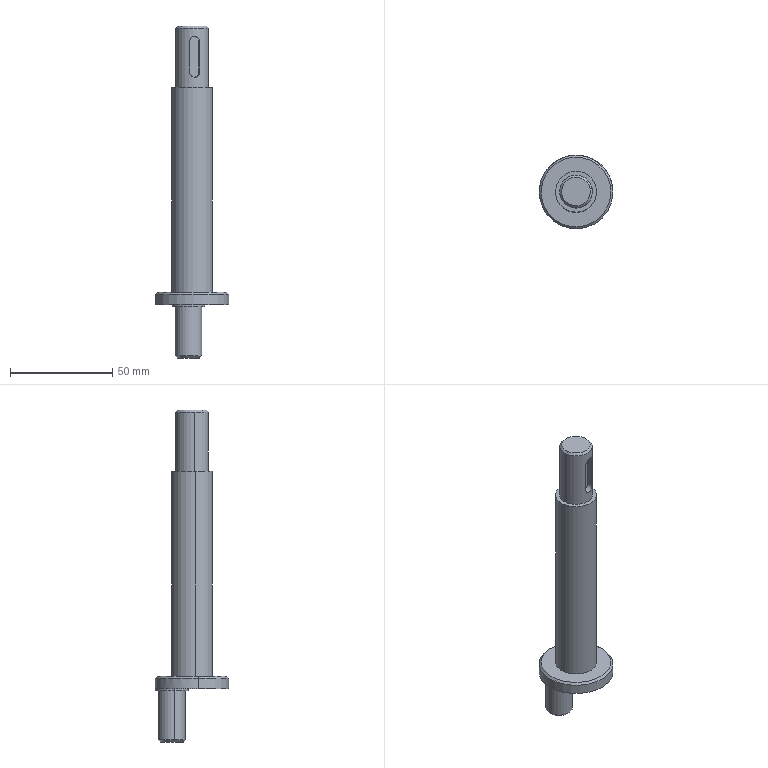Component | SolidWorks | Part5Crankshaft-1 | 1 solid | 27 faces | box 36 x 36 x 162 mm | volume 46703 mm3 | cylinder 12 | plane 9 | cone 6 | commonest cylinder face diameters 16 x4 13 x2 20 x2 36 x2 5 x2
build123d program:
from build123d import *

# Parameters (mm, degrees)
SKETCH1_W           = 30
SKETCH1_H           = 8
SKETCH2_R           = 8
BOSS_EXTRUDE1_DEPTH = 1
SKETCH3_R           = 6.5
BOSS_EXTRUDE2_DEPTH = 25
CHAMFER1_SIZE       = 1
CHAMFER2_SIZE       = 1
CHAMFER3_SIZE       = 1
CUT_EXTRUDE1_DEPTH  = 3


with BuildPart() as part:
    # Sketch1 → Revolve1 (revolve)
    with BuildSketch(Plane.XY, mode=Mode.PRIVATE) as revolve1_sk:
        with Locations((-66, 4)):
            Rectangle(SKETCH1_W, SKETCH1_H)
        Polygon((-51, 8), (-51, 0), (49, 0), (49, 10), (-51, 10), align=None)
        Polygon((49, 10), (49, 0), (55, 0), (55, 18), (49, 18), align=None)
    revolve(revolve1_sk.sketch.rotate(Axis((-81, 0, 0), (1, 0, 0)), 90), axis=Axis((-81, 0, 0), (1, 0, 0)))

    # Sketch2 → Boss-Extrude1 (add)
    with BuildSketch(Plane(origin=(55, 0, 0), x_dir=(0, 0, -1), z_dir=(1, 0, 0))):
        with Locations(Location((0, -10, 0), (0, 0, 270))):
            Circle(SKETCH2_R)
    extrude(amount=BOSS_EXTRUDE1_DEPTH)

    # Sketch3 → Boss-Extrude2 (add)
    with BuildSketch(Plane(origin=(56, 0, 0), x_dir=(0, 0, -1), z_dir=(1, 0, 0))):
        with Locations((0, -10)):
            Circle(SKETCH3_R)
    extrude(amount=BOSS_EXTRUDE2_DEPTH)

    # Chamfer1
    chamfer1_edges = [part.edges().sort_by_distance(p)[0] for p in [
        (81, -10, 6.5),
    ]]
    chamfer(chamfer1_edges, length=CHAMFER1_SIZE)

    # Chamfer2
    chamfer2_edges = [part.edges().sort_by_distance(p)[0] for p in [
        (49, 0, -18),
    ]]
    chamfer(chamfer2_edges, length=CHAMFER2_SIZE)

    # Chamfer3
    chamfer3_edges = [part.edges().sort_by_distance(p)[0] for p in [
        (-81, 0, -8),
    ]]
    chamfer(chamfer3_edges, length=CHAMFER3_SIZE)

    # Sketch6 → Cut-Extrude1 (cut)
    with BuildSketch(Plane(origin=(0, 8, 0), x_dir=(1, 0, 0), z_dir=(0, 1, 0))):
        with BuildLine():
            Line((-73.5, 2.5), (-58.5, 2.5))
            ThreePointArc((-58.5, 2.5), (-56, 0), (-58.5, -2.5))
            Line((-58.5, -2.5), (-73.5, -2.5))
            ThreePointArc((-73.5, -2.5), (-76, 0), (-73.5, 2.5))
        make_face()
    extrude(amount=-CUT_EXTRUDE1_DEPTH, mode=Mode.SUBTRACT)


solid = part.part

# Placed as in the assembly
solid = solid.moved(Location((-80.719, -28.485, 199), (90, -79.746, -90)))
STEP:
#1=COLOUR_RGB('',0.7922,0.8196,0.9333);
#2=FILL_AREA_STYLE_COLOUR('',#1);
#3=FILL_AREA_STYLE('',(#2));
#4=SURFACE_STYLE_FILL_AREA(#3);
#5=SURFACE_SIDE_STYLE('',(#4));
#6=SURFACE_STYLE_USAGE(.BOTH.,#5);
#7=PRESENTATION_STYLE_ASSIGNMENT((#6));
#8=CARTESIAN_POINT('',(-3.449,-1.171,11.024));
#9=VERTEX_POINT('',#8);
#10=CARTESIAN_POINT('',(-2.907,-1.072,11.024));
#11=VERTEX_POINT('',#10);
#12=CARTESIAN_POINT('',(-3.178,-1.121,11.024));
#13=DIRECTION('',(0.,0.,1.));
#14=DIRECTION('',(-0.984,-0.178,0.));
#15=AXIS2_PLACEMENT_3D('',#12,#13,#14);
#16=CIRCLE('',#15,0.2756);
#17=EDGE_CURVE('',#9,#11,#16,.T.);
#18=ORIENTED_EDGE('',*,*,#17,.F.);
#19=CARTESIAN_POINT('',(-3.488,-1.178,10.984));
#20=VERTEX_POINT('',#19);
#21=CARTESIAN_POINT('',(-3.449,-1.171,11.024));
#22=DIRECTION('',(-0.6958,-0.1259,-0.7071));
#23=VECTOR('',#22,39.37);
#24=LINE('',#21,#23);
#25=EDGE_CURVE('',#9,#20,#24,.T.);
#26=ORIENTED_EDGE('',*,*,#25,.T.);
#27=CARTESIAN_POINT('',(-2.868,-1.065,10.984));
#28=VERTEX_POINT('',#27);
#29=CARTESIAN_POINT('',(-3.178,-1.121,10.984));
#30=DIRECTION('',(-0.,-0.,-1.));
#31=DIRECTION('',(-0.984,-0.178,0.));
#32=AXIS2_PLACEMENT_3D('',#29,#30,#31);
#33=CIRCLE('',#32,0.315);
#34=EDGE_CURVE('',#28,#20,#33,.T.);
#35=ORIENTED_EDGE('',*,*,#34,.F.);
#36=CARTESIAN_POINT('',(-2.907,-1.072,11.024));
#37=DIRECTION('',(0.6958,0.1259,-0.7071));
#38=VECTOR('',#37,39.37);
#39=LINE('',#36,#38);
#40=EDGE_CURVE('',#11,#28,#39,.T.);
#41=ORIENTED_EDGE('',*,*,#40,.F.);
#42=EDGE_LOOP('',(#18,#26,#35,#41));
#43=FACE_OUTER_BOUND('',#42,.T.);
#44=CARTESIAN_POINT('',(-3.178,-1.121,11.024));
#45=DIRECTION('',(-0.,-0.,-1.));
#46=DIRECTION('',(0.984,0.178,0.));
#47=AXIS2_PLACEMENT_3D('',#44,#45,#46);
#48=CONICAL_SURFACE('',#47,0.2756,0.7854);
#49=ADVANCED_FACE('',(#43),#48,.T.);
#50=CARTESIAN_POINT('',(-3.837,-1.241,5.906));
#51=VERTEX_POINT('',#50);
#52=CARTESIAN_POINT('',(-2.519,-1.002,5.906));
#53=VERTEX_POINT('',#52);
#54=CARTESIAN_POINT('',(-3.178,-1.121,5.906));
#55=DIRECTION('',(0.,0.,1.));
#56=DIRECTION('',(0.984,0.178,0.));
#57=AXIS2_PLACEMENT_3D('',#54,#55,#56);
#58=CIRCLE('',#57,0.6693);
#59=EDGE_CURVE('',#51,#53,#58,.T.);
#60=ORIENTED_EDGE('',*,*,#59,.F.);
#61=CARTESIAN_POINT('',(-3.875,-1.248,5.866));
#62=VERTEX_POINT('',#61);
#63=CARTESIAN_POINT('',(-3.837,-1.241,5.906));
#64=DIRECTION('',(-0.6958,-0.1259,-0.7071));
#65=VECTOR('',#64,39.37);
#66=LINE('',#63,#65);
#67=EDGE_CURVE('',#51,#62,#66,.T.);
#68=ORIENTED_EDGE('',*,*,#67,.T.);
#69=CARTESIAN_POINT('',(-2.481,-0.9953,5.866));
#70=VERTEX_POINT('',#69);
#71=CARTESIAN_POINT('',(-3.178,-1.121,5.866));
#72=DIRECTION('',(-0.,-0.,-1.));
#73=DIRECTION('',(0.984,0.178,0.));
#74=AXIS2_PLACEMENT_3D('',#71,#72,#73);
#75=CIRCLE('',#74,0.7087);
#76=EDGE_CURVE('',#70,#62,#75,.T.);
#77=ORIENTED_EDGE('',*,*,#76,.F.);
#78=CARTESIAN_POINT('',(-2.519,-1.002,5.906));
#79=DIRECTION('',(0.6958,0.1259,-0.7071));
#80=VECTOR('',#79,39.37);
#81=LINE('',#78,#80);
#82=EDGE_CURVE('',#53,#70,#81,.T.);
#83=ORIENTED_EDGE('',*,*,#82,.F.);
#84=EDGE_LOOP('',(#60,#68,#77,#83));
#85=FACE_OUTER_BOUND('',#84,.T.);
#86=CARTESIAN_POINT('',(-3.178,-1.121,5.906));
#87=DIRECTION('',(-0.,-0.,-1.));
#88=DIRECTION('',(0.984,0.178,0.));
#89=AXIS2_PLACEMENT_3D('',#86,#87,#88);
#90=CONICAL_SURFACE('',#89,0.6693,0.7854);
#91=ADVANCED_FACE('',(#85),#90,.T.);
#92=CARTESIAN_POINT('',(-3.035,-0.6955,4.646));
#93=VERTEX_POINT('',#92);
#94=CARTESIAN_POINT('',(-3.461,-0.7726,4.646));
#95=VERTEX_POINT('',#94);
#96=CARTESIAN_POINT('',(-3.248,-0.7341,4.646));
#97=DIRECTION('',(-0.,-0.,-1.));
#98=DIRECTION('',(0.984,0.178,0.));
#99=AXIS2_PLACEMENT_3D('',#96,#97,#98);
#100=CIRCLE('',#99,0.2165);
#101=EDGE_CURVE('',#93,#95,#100,.T.);
#102=ORIENTED_EDGE('',*,*,#101,.F.);
#103=CARTESIAN_POINT('',(-2.996,-0.6885,4.685));
#104=VERTEX_POINT('',#103);
#105=CARTESIAN_POINT('',(-3.035,-0.6955,4.646));
#106=DIRECTION('',(0.6958,0.1259,0.7071));
#107=VECTOR('',#106,39.37);
#108=LINE('',#105,#107);
#109=EDGE_CURVE('',#93,#104,#108,.T.);
#110=ORIENTED_EDGE('',*,*,#109,.T.);
#111=CARTESIAN_POINT('',(-3.5,-0.7796,4.685));
#112=VERTEX_POINT('',#111);
#113=CARTESIAN_POINT('',(-3.248,-0.7341,4.685));
#114=DIRECTION('',(0.,0.,1.));
#115=DIRECTION('',(0.984,0.178,0.));
#116=AXIS2_PLACEMENT_3D('',#113,#114,#115);
#117=CIRCLE('',#116,0.2559);
#118=EDGE_CURVE('',#112,#104,#117,.T.);
#119=ORIENTED_EDGE('',*,*,#118,.F.);
#120=CARTESIAN_POINT('',(-3.461,-0.7726,4.646));
#121=DIRECTION('',(-0.6958,-0.1259,0.7071));
#122=VECTOR('',#121,39.37);
#123=LINE('',#120,#122);
#124=EDGE_CURVE('',#95,#112,#123,.T.);
#125=ORIENTED_EDGE('',*,*,#124,.F.);
#126=EDGE_LOOP('',(#102,#110,#119,#125));
#127=FACE_OUTER_BOUND('',#126,.T.);
#128=CARTESIAN_POINT('',(-3.248,-0.7341,4.646));
#129=DIRECTION('',(0.,0.,1.));
#130=DIRECTION('',(-0.984,-0.178,0.));
#131=AXIS2_PLACEMENT_3D('',#128,#129,#130);
#132=CONICAL_SURFACE('',#131,0.2165,0.7854);
#133=ADVANCED_FACE('',(#127),#132,.T.);
#134=ORIENTED_EDGE('',*,*,#118,.T.);
#135=CARTESIAN_POINT('',(-2.996,-0.6885,5.63));
#136=VERTEX_POINT('',#135);
#137=CARTESIAN_POINT('',(-2.996,-0.6885,4.646));
#138=DIRECTION('',(0.,0.,1.));
#139=VECTOR('',#138,39.37);
#140=LINE('',#137,#139);
#141=EDGE_CURVE('',#104,#136,#140,.T.);
#142=ORIENTED_EDGE('',*,*,#141,.T.);
#143=CARTESIAN_POINT('',(-3.5,-0.7796,5.63));
#144=VERTEX_POINT('',#143);
#145=CARTESIAN_POINT('',(-3.248,-0.7341,5.63));
#146=DIRECTION('',(-0.,-0.,-1.));
#147=DIRECTION('',(0.984,0.178,0.));
#148=AXIS2_PLACEMENT_3D('',#145,#146,#147);
#149=CIRCLE('',#148,0.2559);
#150=EDGE_CURVE('',#136,#144,#149,.T.);
#151=ORIENTED_EDGE('',*,*,#150,.T.);
#152=CARTESIAN_POINT('',(-3.5,-0.7796,4.646));
#153=DIRECTION('',(0.,0.,1.));
#154=VECTOR('',#153,39.37);
#155=LINE('',#152,#154);
#156=EDGE_CURVE('',#112,#144,#155,.T.);
#157=ORIENTED_EDGE('',*,*,#156,.F.);
#158=EDGE_LOOP('',(#134,#142,#151,#157));
#159=FACE_OUTER_BOUND('',#158,.T.);
#160=CARTESIAN_POINT('',(-3.248,-0.7341,4.646));
#161=DIRECTION('',(0.,0.,1.));
#162=DIRECTION('',(-0.984,-0.178,0.));
#163=AXIS2_PLACEMENT_3D('',#160,#161,#162);
#164=CYLINDRICAL_SURFACE('',#163,0.2559);
#165=ADVANCED_FACE('',(#159),#164,.T.);
#166=CARTESIAN_POINT('',(-2.938,-0.678,5.63));
#167=VERTEX_POINT('',#166);
#168=CARTESIAN_POINT('',(-3.558,-0.7901,5.63));
#169=VERTEX_POINT('',#168);
#170=CARTESIAN_POINT('',(-3.248,-0.7341,5.63));
#171=DIRECTION('',(-0.,-0.,-1.));
#172=DIRECTION('',(0.984,0.178,0.));
#173=AXIS2_PLACEMENT_3D('',#170,#171,#172);
#174=CIRCLE('',#173,0.315);
#175=EDGE_CURVE('',#167,#169,#174,.T.);
#176=ORIENTED_EDGE('',*,*,#175,.F.);
#177=CARTESIAN_POINT('',(-2.938,-0.678,5.669));
#178=VERTEX_POINT('',#177);
#179=CARTESIAN_POINT('',(-2.938,-0.678,5.63));
#180=DIRECTION('',(0.,0.,1.));
#181=VECTOR('',#180,39.37);
#182=LINE('',#179,#181);
#183=EDGE_CURVE('',#167,#178,#182,.T.);
#184=ORIENTED_EDGE('',*,*,#183,.T.);
#185=CARTESIAN_POINT('',(-3.558,-0.7901,5.669));
#186=VERTEX_POINT('',#185);
#187=CARTESIAN_POINT('',(-3.248,-0.7341,5.669));
#188=DIRECTION('',(-0.,-0.,-1.));
#189=DIRECTION('',(0.984,0.178,0.));
#190=AXIS2_PLACEMENT_3D('',#187,#188,#189);
#191=CIRCLE('',#190,0.315);
#192=EDGE_CURVE('',#178,#186,#191,.T.);
#193=ORIENTED_EDGE('',*,*,#192,.T.);
#194=CARTESIAN_POINT('',(-3.558,-0.7901,5.63));
#195=DIRECTION('',(0.,0.,1.));
#196=VECTOR('',#195,39.37);
#197=LINE('',#194,#196);
#198=EDGE_CURVE('',#169,#186,#197,.T.);
#199=ORIENTED_EDGE('',*,*,#198,.F.);
#200=EDGE_LOOP('',(#176,#184,#193,#199));
#201=FACE_OUTER_BOUND('',#200,.T.);
#202=CARTESIAN_POINT('',(-3.248,-0.7341,5.63));
#203=DIRECTION('',(0.,0.,1.));
#204=DIRECTION('',(-0.984,-0.178,0.));
#205=AXIS2_PLACEMENT_3D('',#202,#203,#204);
#206=CYLINDRICAL_SURFACE('',#205,0.315);
#207=ADVANCED_FACE('',(#201),#206,.T.);
#208=CARTESIAN_POINT('',(-3.222,-1.433,10.138));
#209=VERTEX_POINT('',#208);
#210=CARTESIAN_POINT('',(-3.028,-1.398,10.138));
#211=VERTEX_POINT('',#210);
#212=CARTESIAN_POINT('',(-3.222,-1.433,10.138));
#213=CARTESIAN_POINT('',(-3.222,-1.433,10.131));
#214=CARTESIAN_POINT('',(-3.221,-1.433,10.125));
#215=CARTESIAN_POINT('',(-3.218,-1.434,10.112));
#216=CARTESIAN_POINT('',(-3.216,-1.434,10.106));
#217=CARTESIAN_POINT('',(-3.211,-1.435,10.094));
#218=CARTESIAN_POINT('',(-3.208,-1.435,10.088));
#219=CARTESIAN_POINT('',(-3.201,-1.436,10.078));
#220=CARTESIAN_POINT('',(-3.196,-1.436,10.073));
#221=CARTESIAN_POINT('',(-3.182,-1.437,10.059));
#222=CARTESIAN_POINT('',(-3.171,-1.437,10.052));
#223=CARTESIAN_POINT('',(-3.154,-1.436,10.044));
#224=CARTESIAN_POINT('',(-3.147,-1.435,10.043));
#225=CARTESIAN_POINT('',(-3.135,-1.434,10.04));
#226=CARTESIAN_POINT('',(-3.128,-1.433,10.039));
#227=CARTESIAN_POINT('',(-3.116,-1.43,10.039));
#228=CARTESIAN_POINT('',(-3.109,-1.429,10.04));
#229=CARTESIAN_POINT('',(-3.097,-1.426,10.043));
#230=CARTESIAN_POINT('',(-3.091,-1.424,10.044));
#231=CARTESIAN_POINT('',(-3.079,-1.421,10.049));
#232=CARTESIAN_POINT('',(-3.074,-1.419,10.052));
#233=CARTESIAN_POINT('',(-3.064,-1.415,10.06));
#234=CARTESIAN_POINT('',(-3.059,-1.413,10.064));
#235=CARTESIAN_POINT('',(-3.05,-1.41,10.073));
#236=CARTESIAN_POINT('',(-3.047,-1.408,10.078));
#237=CARTESIAN_POINT('',(-3.04,-1.405,10.088));
#238=CARTESIAN_POINT('',(-3.037,-1.403,10.094));
#239=CARTESIAN_POINT('',(-3.033,-1.401,10.106));
#240=CARTESIAN_POINT('',(-3.031,-1.4,10.112));
#241=CARTESIAN_POINT('',(-3.028,-1.399,10.125));
#242=CARTESIAN_POINT('',(-3.028,-1.398,10.131));
#243=CARTESIAN_POINT('',(-3.028,-1.398,10.138));
#244=B_SPLINE_CURVE_WITH_KNOTS('',3,(#212,#213,#214,#215,#216,#217,#218,#219,#220,#221,#222,#223,#224,#225,#226,#227,#228,#229,#230,#231,#232,#233,#234,#235,#236,#237,#238,#239,#240,#241,#242,#243),.UNSPECIFIED.,.F.,.F.,(4,2,2,2,2,2,2,2,2,2,2,2,2,2,2,4),(0.,0.0004914,0.0009828,0.001474,0.001966,0.002949,0.00344,0.003931,0.004423,0.004914,0.005406,0.005897,0.006388,0.00688,0.007371,0.007863),.UNSPECIFIED.);
#245=EDGE_CURVE('',#209,#211,#244,.T.);
#246=ORIENTED_EDGE('',*,*,#245,.F.);
#247=CARTESIAN_POINT('',(-3.222,-1.433,10.728));
#248=VERTEX_POINT('',#247);
#249=CARTESIAN_POINT('',(-3.222,-1.433,11.024));
#250=DIRECTION('',(-0.,-0.,-1.));
#251=VECTOR('',#250,39.37);
#252=LINE('',#249,#251);
#253=EDGE_CURVE('',#248,#209,#252,.T.);
#254=ORIENTED_EDGE('',*,*,#253,.F.);
#255=CARTESIAN_POINT('',(-3.028,-1.398,10.728));
#256=VERTEX_POINT('',#255);
#257=CARTESIAN_POINT('',(-3.028,-1.398,10.728));
#258=CARTESIAN_POINT('',(-3.028,-1.398,10.735));
#259=CARTESIAN_POINT('',(-3.028,-1.399,10.741));
#260=CARTESIAN_POINT('',(-3.031,-1.4,10.754));
#261=CARTESIAN_POINT('',(-3.033,-1.401,10.76));
#262=CARTESIAN_POINT('',(-3.037,-1.403,10.772));
#263=CARTESIAN_POINT('',(-3.04,-1.405,10.778));
#264=CARTESIAN_POINT('',(-3.047,-1.408,10.788));
#265=CARTESIAN_POINT('',(-3.05,-1.41,10.793));
#266=CARTESIAN_POINT('',(-3.063,-1.415,10.807));
#267=CARTESIAN_POINT('',(-3.074,-1.419,10.814));
#268=CARTESIAN_POINT('',(-3.091,-1.424,10.822));
#269=CARTESIAN_POINT('',(-3.097,-1.426,10.824));
#270=CARTESIAN_POINT('',(-3.109,-1.429,10.826));
#271=CARTESIAN_POINT('',(-3.115,-1.43,10.827));
#272=CARTESIAN_POINT('',(-3.128,-1.433,10.827));
#273=CARTESIAN_POINT('',(-3.135,-1.434,10.826));
#274=CARTESIAN_POINT('',(-3.147,-1.435,10.824));
#275=CARTESIAN_POINT('',(-3.153,-1.436,10.822));
#276=CARTESIAN_POINT('',(-3.165,-1.436,10.817));
#277=CARTESIAN_POINT('',(-3.171,-1.436,10.814));
#278=CARTESIAN_POINT('',(-3.182,-1.436,10.807));
#279=CARTESIAN_POINT('',(-3.187,-1.436,10.802));
#280=CARTESIAN_POINT('',(-3.196,-1.436,10.793));
#281=CARTESIAN_POINT('',(-3.201,-1.436,10.789));
#282=CARTESIAN_POINT('',(-3.208,-1.435,10.778));
#283=CARTESIAN_POINT('',(-3.211,-1.435,10.772));
#284=CARTESIAN_POINT('',(-3.216,-1.434,10.76));
#285=CARTESIAN_POINT('',(-3.218,-1.434,10.754));
#286=CARTESIAN_POINT('',(-3.221,-1.433,10.741));
#287=CARTESIAN_POINT('',(-3.222,-1.433,10.735));
#288=CARTESIAN_POINT('',(-3.222,-1.433,10.728));
#289=B_SPLINE_CURVE_WITH_KNOTS('',3,(#257,#258,#259,#260,#261,#262,#263,#264,#265,#266,#267,#268,#269,#270,#271,#272,#273,#274,#275,#276,#277,#278,#279,#280,#281,#282,#283,#284,#285,#286,#287,#288),.UNSPECIFIED.,.F.,.F.,(4,2,2,2,2,2,2,2,2,2,2,2,2,2,2,4),(0.,0.0004914,0.0009828,0.001474,0.001966,0.002949,0.00344,0.003931,0.004423,0.004914,0.005406,0.005897,0.006388,0.00688,0.007371,0.007863),.UNSPECIFIED.);
#290=EDGE_CURVE('',#256,#248,#289,.T.);
#291=ORIENTED_EDGE('',*,*,#290,.F.);
#292=CARTESIAN_POINT('',(-3.028,-1.398,11.024));
#293=DIRECTION('',(0.,0.,1.));
#294=VECTOR('',#293,39.37);
#295=LINE('',#292,#294);
#296=EDGE_CURVE('',#211,#256,#295,.T.);
#297=ORIENTED_EDGE('',*,*,#296,.F.);
#298=EDGE_LOOP('',(#246,#254,#291,#297));
#299=FACE_BOUND('',#298,.T.);
#300=CARTESIAN_POINT('',(-3.488,-1.178,9.843));
#301=VERTEX_POINT('',#300);
#302=CARTESIAN_POINT('',(-2.868,-1.065,9.843));
#303=VERTEX_POINT('',#302);
#304=CARTESIAN_POINT('',(-3.178,-1.121,9.843));
#305=DIRECTION('',(0.,0.,1.));
#306=DIRECTION('',(-0.984,-0.178,0.));
#307=AXIS2_PLACEMENT_3D('',#304,#305,#306);
#308=CIRCLE('',#307,0.315);
#309=EDGE_CURVE('',#301,#303,#308,.T.);
#310=ORIENTED_EDGE('',*,*,#309,.T.);
#311=CARTESIAN_POINT('',(-2.868,-1.065,11.024));
#312=DIRECTION('',(0.,0.,1.));
#313=VECTOR('',#312,39.37);
#314=LINE('',#311,#313);
#315=EDGE_CURVE('',#303,#28,#314,.T.);
#316=ORIENTED_EDGE('',*,*,#315,.T.);
#317=ORIENTED_EDGE('',*,*,#34,.T.);
#318=CARTESIAN_POINT('',(-3.488,-1.178,11.024));
#319=DIRECTION('',(0.,0.,1.));
#320=VECTOR('',#319,39.37);
#321=LINE('',#318,#320);
#322=EDGE_CURVE('',#301,#20,#321,.T.);
#323=ORIENTED_EDGE('',*,*,#322,.F.);
#324=EDGE_LOOP('',(#310,#316,#317,#323));
#325=FACE_OUTER_BOUND('',#324,.T.);
#326=CARTESIAN_POINT('',(-3.178,-1.121,11.024));
#327=DIRECTION('',(0.,0.,1.));
#328=DIRECTION('',(-0.984,-0.178,0.));
#329=AXIS2_PLACEMENT_3D('',#326,#327,#328);
#330=CYLINDRICAL_SURFACE('',#329,0.315);
#331=ADVANCED_FACE('',(#299,#325),#330,.T.);
#332=CARTESIAN_POINT('',(-3.565,-1.192,5.906));
#333=VERTEX_POINT('',#332);
#334=CARTESIAN_POINT('',(-2.79,-1.051,5.906));
#335=VERTEX_POINT('',#334);
#336=CARTESIAN_POINT('',(-3.178,-1.121,5.906));
#337=DIRECTION('',(0.,0.,1.));
#338=DIRECTION('',(-0.984,-0.178,0.));
#339=AXIS2_PLACEMENT_3D('',#336,#337,#338);
#340=CIRCLE('',#339,0.3937);
#341=EDGE_CURVE('',#333,#335,#340,.T.);
#342=ORIENTED_EDGE('',*,*,#341,.T.);
#343=CARTESIAN_POINT('',(-2.79,-1.051,9.843));
#344=VERTEX_POINT('',#343);
#345=CARTESIAN_POINT('',(-2.79,-1.051,11.024));
#346=DIRECTION('',(0.,0.,1.));
#347=VECTOR('',#346,39.37);
#348=LINE('',#345,#347);
#349=EDGE_CURVE('',#335,#344,#348,.T.);
#350=ORIENTED_EDGE('',*,*,#349,.T.);
#351=CARTESIAN_POINT('',(-3.565,-1.192,9.843));
#352=VERTEX_POINT('',#351);
#353=CARTESIAN_POINT('',(-3.178,-1.121,9.843));
#354=DIRECTION('',(0.,0.,1.));
#355=DIRECTION('',(-0.984,-0.178,0.));
#356=AXIS2_PLACEMENT_3D('',#353,#354,#355);
#357=CIRCLE('',#356,0.3937);
#358=EDGE_CURVE('',#352,#344,#357,.T.);
#359=ORIENTED_EDGE('',*,*,#358,.F.);
#360=CARTESIAN_POINT('',(-3.565,-1.192,11.024));
#361=DIRECTION('',(0.,0.,1.));
#362=VECTOR('',#361,39.37);
#363=LINE('',#360,#362);
#364=EDGE_CURVE('',#333,#352,#363,.T.);
#365=ORIENTED_EDGE('',*,*,#364,.F.);
#366=EDGE_LOOP('',(#342,#350,#359,#365));
#367=FACE_OUTER_BOUND('',#366,.T.);
#368=CARTESIAN_POINT('',(-3.178,-1.121,11.024));
#369=DIRECTION('',(0.,0.,1.));
#370=DIRECTION('',(-0.984,-0.178,0.));
#371=AXIS2_PLACEMENT_3D('',#368,#369,#370);
#372=CYLINDRICAL_SURFACE('',#371,0.3937);
#373=ADVANCED_FACE('',(#367),#372,.T.);
#374=CARTESIAN_POINT('',(-3.875,-1.248,5.669));
#375=VERTEX_POINT('',#374);
#376=CARTESIAN_POINT('',(-2.481,-0.9953,5.669));
#377=VERTEX_POINT('',#376);
#378=CARTESIAN_POINT('',(-3.178,-1.121,5.669));
#379=DIRECTION('',(0.,0.,1.));
#380=DIRECTION('',(-0.984,-0.178,0.));
#381=AXIS2_PLACEMENT_3D('',#378,#379,#380);
#382=CIRCLE('',#381,0.7087);
#383=EDGE_CURVE('',#375,#377,#382,.T.);
#384=ORIENTED_EDGE('',*,*,#383,.T.);
#385=CARTESIAN_POINT('',(-2.481,-0.9953,11.024));
#386=DIRECTION('',(0.,0.,1.));
#387=VECTOR('',#386,39.37);
#388=LINE('',#385,#387);
#389=EDGE_CURVE('',#377,#70,#388,.T.);
#390=ORIENTED_EDGE('',*,*,#389,.T.);
#391=ORIENTED_EDGE('',*,*,#76,.T.);
#392=CARTESIAN_POINT('',(-3.875,-1.248,11.024));
#393=DIRECTION('',(0.,0.,1.));
#394=VECTOR('',#393,39.37);
#395=LINE('',#392,#394);
#396=EDGE_CURVE('',#375,#62,#395,.T.);
#397=ORIENTED_EDGE('',*,*,#396,.F.);
#398=EDGE_LOOP('',(#384,#390,#391,#397));
#399=FACE_OUTER_BOUND('',#398,.T.);
#400=CARTESIAN_POINT('',(-3.178,-1.121,11.024));
#401=DIRECTION('',(0.,0.,1.));
#402=DIRECTION('',(-0.984,-0.178,0.));
#403=AXIS2_PLACEMENT_3D('',#400,#401,#402);
#404=CYLINDRICAL_SURFACE('',#403,0.7087);
#405=ADVANCED_FACE('',(#399),#404,.T.);
#406=CARTESIAN_POINT('',(-3.178,-1.121,11.024));
#407=DIRECTION('',(0.,0.,1.));
#408=DIRECTION('',(-0.984,-0.178,0.));
#409=AXIS2_PLACEMENT_3D('',#406,#407,#408);
#410=CIRCLE('',#409,0.2756);
#411=EDGE_CURVE('',#11,#9,#410,.T.);
#412=ORIENTED_EDGE('',*,*,#411,.T.);
#413=ORIENTED_EDGE('',*,*,#17,.T.);
#414=EDGE_LOOP('',(#412,#413));
#415=FACE_OUTER_BOUND('',#414,.T.);
#416=CARTESIAN_POINT('',(-3.178,-1.121,11.024));
#417=DIRECTION('',(0.,0.,1.));
#418=DIRECTION('',(-0.984,-0.178,0.));
#419=AXIS2_PLACEMENT_3D('',#416,#417,#418);
#420=PLANE('',#419);
#421=ADVANCED_FACE('',(#415),#420,.T.);
#422=CARTESIAN_POINT('',(-3.304,-0.4241,5.669));
#423=VERTEX_POINT('',#422);
#424=CARTESIAN_POINT('',(-3.178,-1.121,5.669));
#425=DIRECTION('',(0.,0.,1.));
#426=DIRECTION('',(-0.984,-0.178,0.));
#427=AXIS2_PLACEMENT_3D('',#424,#425,#426);
#428=CIRCLE('',#427,0.7087);
#429=EDGE_CURVE('',#423,#375,#428,.T.);
#430=ORIENTED_EDGE('',*,*,#429,.F.);
#431=CARTESIAN_POINT('',(-3.248,-0.7341,5.669));
#432=DIRECTION('',(-0.,-0.,-1.));
#433=DIRECTION('',(0.984,0.178,0.));
#434=AXIS2_PLACEMENT_3D('',#431,#432,#433);
#435=CIRCLE('',#434,0.315);
#436=EDGE_CURVE('',#186,#423,#435,.T.);
#437=ORIENTED_EDGE('',*,*,#436,.F.);
#438=ORIENTED_EDGE('',*,*,#192,.F.);
#439=CARTESIAN_POINT('',(-3.248,-0.7341,5.669));
#440=DIRECTION('',(-0.,-0.,-1.));
#441=DIRECTION('',(0.984,0.178,0.));
#442=AXIS2_PLACEMENT_3D('',#439,#440,#441);
#443=CIRCLE('',#442,0.315);
#444=EDGE_CURVE('',#423,#178,#443,.T.);
#445=ORIENTED_EDGE('',*,*,#444,.F.);
#446=CARTESIAN_POINT('',(-3.178,-1.121,5.669));
#447=DIRECTION('',(0.,0.,1.));
#448=DIRECTION('',(-0.984,-0.178,0.));
#449=AXIS2_PLACEMENT_3D('',#446,#447,#448);
#450=CIRCLE('',#449,0.7087);
#451=EDGE_CURVE('',#377,#423,#450,.T.);
#452=ORIENTED_EDGE('',*,*,#451,.F.);
#453=ORIENTED_EDGE('',*,*,#383,.F.);
#454=EDGE_LOOP('',(#430,#437,#438,#445,#452,#453));
#455=FACE_OUTER_BOUND('',#454,.T.);
#456=CARTESIAN_POINT('',(-3.178,-1.121,5.669));
#457=DIRECTION('',(-0.,-0.,-1.));
#458=DIRECTION('',(0.984,0.178,-0.));
#459=AXIS2_PLACEMENT_3D('',#456,#457,#458);
#460=PLANE('',#459);
#461=ADVANCED_FACE('',(#455),#460,.T.);
#462=ORIENTED_EDGE('',*,*,#389,.F.);
#463=ORIENTED_EDGE('',*,*,#451,.T.);
#464=ORIENTED_EDGE('',*,*,#429,.T.);
#465=ORIENTED_EDGE('',*,*,#396,.T.);
#466=CARTESIAN_POINT('',(-3.178,-1.121,5.866));
#467=DIRECTION('',(-0.,-0.,-1.));
#468=DIRECTION('',(0.984,0.178,0.));
#469=AXIS2_PLACEMENT_3D('',#466,#467,#468);
#470=CIRCLE('',#469,0.7087);
#471=EDGE_CURVE('',#62,#70,#470,.T.);
#472=ORIENTED_EDGE('',*,*,#471,.T.);
#473=EDGE_LOOP('',(#462,#463,#464,#465,#472));
#474=FACE_OUTER_BOUND('',#473,.T.);
#475=CARTESIAN_POINT('',(-3.178,-1.121,11.024));
#476=DIRECTION('',(0.,0.,1.));
#477=DIRECTION('',(-0.984,-0.178,0.));
#478=AXIS2_PLACEMENT_3D('',#475,#476,#477);
#479=CYLINDRICAL_SURFACE('',#478,0.7087);
#480=ADVANCED_FACE('',(#474),#479,.T.);
#481=CARTESIAN_POINT('',(-3.178,-1.121,5.906));
#482=DIRECTION('',(0.,0.,1.));
#483=DIRECTION('',(0.984,0.178,0.));
#484=AXIS2_PLACEMENT_3D('',#481,#482,#483);
#485=CIRCLE('',#484,0.6693);
#486=EDGE_CURVE('',#53,#51,#485,.T.);
#487=ORIENTED_EDGE('',*,*,#486,.T.);
#488=ORIENTED_EDGE('',*,*,#59,.T.);
#489=EDGE_LOOP('',(#487,#488));
#490=FACE_OUTER_BOUND('',#489,.T.);
#491=ORIENTED_EDGE('',*,*,#341,.F.);
#492=CARTESIAN_POINT('',(-3.178,-1.121,5.906));
#493=DIRECTION('',(0.,0.,1.));
#494=DIRECTION('',(-0.984,-0.178,0.));
#495=AXIS2_PLACEMENT_3D('',#492,#493,#494);
#496=CIRCLE('',#495,0.3937);
#497=EDGE_CURVE('',#335,#333,#496,.T.);
#498=ORIENTED_EDGE('',*,*,#497,.F.);
#499=EDGE_LOOP('',(#491,#498));
#500=FACE_BOUND('',#499,.T.);
#501=CARTESIAN_POINT('',(-3.178,-1.121,5.906));
#502=DIRECTION('',(-0.,-0.,-1.));
#503=DIRECTION('',(0.984,0.178,-0.));
#504=AXIS2_PLACEMENT_3D('',#501,#502,#503);
#505=PLANE('',#504);
#506=ADVANCED_FACE('',(#490,#500),#505,.F.);
#507=ORIENTED_EDGE('',*,*,#349,.F.);
#508=ORIENTED_EDGE('',*,*,#497,.T.);
#509=ORIENTED_EDGE('',*,*,#364,.T.);
#510=CARTESIAN_POINT('',(-3.178,-1.121,9.843));
#511=DIRECTION('',(0.,0.,1.));
#512=DIRECTION('',(-0.984,-0.178,0.));
#513=AXIS2_PLACEMENT_3D('',#510,#511,#512);
#514=CIRCLE('',#513,0.3937);
#515=EDGE_CURVE('',#344,#352,#514,.T.);
#516=ORIENTED_EDGE('',*,*,#515,.F.);
#517=EDGE_LOOP('',(#507,#508,#509,#516));
#518=FACE_OUTER_BOUND('',#517,.T.);
#519=CARTESIAN_POINT('',(-3.178,-1.121,11.024));
#520=DIRECTION('',(0.,0.,1.));
#521=DIRECTION('',(-0.984,-0.178,0.));
#522=AXIS2_PLACEMENT_3D('',#519,#520,#521);
#523=CYLINDRICAL_SURFACE('',#522,0.3937);
#524=ADVANCED_FACE('',(#518),#523,.T.);
#525=ORIENTED_EDGE('',*,*,#309,.F.);
#526=CARTESIAN_POINT('',(-3.178,-1.121,9.843));
#527=DIRECTION('',(0.,0.,1.));
#528=DIRECTION('',(-0.984,-0.178,0.));
#529=AXIS2_PLACEMENT_3D('',#526,#527,#528);
#530=CIRCLE('',#529,0.315);
#531=EDGE_CURVE('',#303,#301,#530,.T.);
#532=ORIENTED_EDGE('',*,*,#531,.F.);
#533=EDGE_LOOP('',(#525,#532));
#534=FACE_BOUND('',#533,.T.);
#535=ORIENTED_EDGE('',*,*,#358,.T.);
#536=ORIENTED_EDGE('',*,*,#515,.T.);
#537=EDGE_LOOP('',(#535,#536));
#538=FACE_OUTER_BOUND('',#537,.T.);
#539=CARTESIAN_POINT('',(-3.178,-1.121,9.843));
#540=DIRECTION('',(-0.,-0.,-1.));
#541=DIRECTION('',(0.984,0.178,-0.));
#542=AXIS2_PLACEMENT_3D('',#539,#540,#541);
#543=PLANE('',#542);
#544=ADVANCED_FACE('',(#534,#538),#543,.F.);
#545=ORIENTED_EDGE('',*,*,#315,.F.);
#546=ORIENTED_EDGE('',*,*,#531,.T.);
#547=ORIENTED_EDGE('',*,*,#322,.T.);
#548=CARTESIAN_POINT('',(-3.178,-1.121,10.984));
#549=DIRECTION('',(-0.,-0.,-1.));
#550=DIRECTION('',(-0.984,-0.178,0.));
#551=AXIS2_PLACEMENT_3D('',#548,#549,#550);
#552=CIRCLE('',#551,0.315);
#553=EDGE_CURVE('',#20,#28,#552,.T.);
#554=ORIENTED_EDGE('',*,*,#553,.T.);
#555=EDGE_LOOP('',(#545,#546,#547,#554));
#556=FACE_OUTER_BOUND('',#555,.T.);
#557=CARTESIAN_POINT('',(-3.178,-1.121,11.024));
#558=DIRECTION('',(0.,0.,1.));
#559=DIRECTION('',(-0.984,-0.178,0.));
#560=AXIS2_PLACEMENT_3D('',#557,#558,#559);
#561=CYLINDRICAL_SURFACE('',#560,0.315);
#562=ADVANCED_FACE('',(#556),#561,.T.);
#563=ORIENTED_EDGE('',*,*,#183,.F.);
#564=CARTESIAN_POINT('',(-3.248,-0.7341,5.63));
#565=DIRECTION('',(-0.,-0.,-1.));
#566=DIRECTION('',(0.984,0.178,0.));
#567=AXIS2_PLACEMENT_3D('',#564,#565,#566);
#568=CIRCLE('',#567,0.315);
#569=EDGE_CURVE('',#169,#167,#568,.T.);
#570=ORIENTED_EDGE('',*,*,#569,.F.);
#571=ORIENTED_EDGE('',*,*,#198,.T.);
#572=ORIENTED_EDGE('',*,*,#436,.T.);
#573=ORIENTED_EDGE('',*,*,#444,.T.);
#574=EDGE_LOOP('',(#563,#570,#571,#572,#573));
#575=FACE_OUTER_BOUND('',#574,.T.);
#576=CARTESIAN_POINT('',(-3.248,-0.7341,5.63));
#577=DIRECTION('',(0.,0.,1.));
#578=DIRECTION('',(-0.984,-0.178,0.));
#579=AXIS2_PLACEMENT_3D('',#576,#577,#578);
#580=CYLINDRICAL_SURFACE('',#579,0.315);
#581=ADVANCED_FACE('',(#575),#580,.T.);
#582=CARTESIAN_POINT('',(-3.248,-0.7341,5.63));
#583=DIRECTION('',(-0.,-0.,-1.));
#584=DIRECTION('',(0.984,0.178,0.));
#585=AXIS2_PLACEMENT_3D('',#582,#583,#584);
#586=CIRCLE('',#585,0.2559);
#587=EDGE_CURVE('',#144,#136,#586,.T.);
#588=ORIENTED_EDGE('',*,*,#587,.F.);
#589=ORIENTED_EDGE('',*,*,#150,.F.);
#590=EDGE_LOOP('',(#588,#589));
#591=FACE_BOUND('',#590,.T.);
#592=ORIENTED_EDGE('',*,*,#569,.T.);
#593=ORIENTED_EDGE('',*,*,#175,.T.);
#594=EDGE_LOOP('',(#592,#593));
#595=FACE_OUTER_BOUND('',#594,.T.);
#596=CARTESIAN_POINT('',(-3.248,-0.7341,5.63));
#597=DIRECTION('',(-0.,-0.,-1.));
#598=DIRECTION('',(0.984,0.178,-0.));
#599=AXIS2_PLACEMENT_3D('',#596,#597,#598);
#600=PLANE('',#599);
#601=ADVANCED_FACE('',(#591,#595),#600,.T.);
#602=ORIENTED_EDGE('',*,*,#141,.F.);
#603=CARTESIAN_POINT('',(-3.248,-0.7341,4.685));
#604=DIRECTION('',(0.,0.,1.));
#605=DIRECTION('',(0.984,0.178,0.));
#606=AXIS2_PLACEMENT_3D('',#603,#604,#605);
#607=CIRCLE('',#606,0.2559);
#608=EDGE_CURVE('',#104,#112,#607,.T.);
#609=ORIENTED_EDGE('',*,*,#608,.T.);
#610=ORIENTED_EDGE('',*,*,#156,.T.);
#611=ORIENTED_EDGE('',*,*,#587,.T.);
#612=EDGE_LOOP('',(#602,#609,#610,#611));
#613=FACE_OUTER_BOUND('',#612,.T.);
#614=CARTESIAN_POINT('',(-3.248,-0.7341,4.646));
#615=DIRECTION('',(0.,0.,1.));
#616=DIRECTION('',(-0.984,-0.178,0.));
#617=AXIS2_PLACEMENT_3D('',#614,#615,#616);
#618=CYLINDRICAL_SURFACE('',#617,0.2559);
#619=ADVANCED_FACE('',(#613),#618,.T.);
#620=CARTESIAN_POINT('',(-3.248,-0.7341,4.646));
#621=DIRECTION('',(-0.,-0.,-1.));
#622=DIRECTION('',(0.984,0.178,0.));
#623=AXIS2_PLACEMENT_3D('',#620,#621,#622);
#624=CIRCLE('',#623,0.2165);
#625=EDGE_CURVE('',#95,#93,#624,.T.);
#626=ORIENTED_EDGE('',*,*,#625,.T.);
#627=ORIENTED_EDGE('',*,*,#101,.T.);
#628=EDGE_LOOP('',(#626,#627));
#629=FACE_OUTER_BOUND('',#628,.T.);
#630=CARTESIAN_POINT('',(-3.248,-0.7341,4.646));
#631=DIRECTION('',(-0.,-0.,-1.));
#632=DIRECTION('',(0.984,0.178,-0.));
#633=AXIS2_PLACEMENT_3D('',#630,#631,#632);
#634=PLANE('',#633);
#635=ADVANCED_FACE('',(#629),#634,.T.);
#636=ORIENTED_EDGE('',*,*,#109,.F.);
#637=ORIENTED_EDGE('',*,*,#625,.F.);
#638=ORIENTED_EDGE('',*,*,#124,.T.);
#639=ORIENTED_EDGE('',*,*,#608,.F.);
#640=EDGE_LOOP('',(#636,#637,#638,#639));
#641=FACE_OUTER_BOUND('',#640,.T.);
#642=CARTESIAN_POINT('',(-3.248,-0.7341,4.646));
#643=DIRECTION('',(0.,0.,1.));
#644=DIRECTION('',(-0.984,-0.178,0.));
#645=AXIS2_PLACEMENT_3D('',#642,#643,#644);
#646=CONICAL_SURFACE('',#645,0.2165,0.7854);
#647=ADVANCED_FACE('',(#641),#646,.T.);
#648=ORIENTED_EDGE('',*,*,#67,.F.);
#649=ORIENTED_EDGE('',*,*,#486,.F.);
#650=ORIENTED_EDGE('',*,*,#82,.T.);
#651=ORIENTED_EDGE('',*,*,#471,.F.);
#652=EDGE_LOOP('',(#648,#649,#650,#651));
#653=FACE_OUTER_BOUND('',#652,.T.);
#654=CARTESIAN_POINT('',(-3.178,-1.121,5.906));
#655=DIRECTION('',(-0.,-0.,-1.));
#656=DIRECTION('',(0.984,0.178,0.));
#657=AXIS2_PLACEMENT_3D('',#654,#655,#656);
#658=CONICAL_SURFACE('',#657,0.6693,0.7854);
#659=ADVANCED_FACE('',(#653),#658,.T.);
#660=ORIENTED_EDGE('',*,*,#25,.F.);
#661=ORIENTED_EDGE('',*,*,#411,.F.);
#662=ORIENTED_EDGE('',*,*,#40,.T.);
#663=ORIENTED_EDGE('',*,*,#553,.F.);
#664=EDGE_LOOP('',(#660,#661,#662,#663));
#665=FACE_OUTER_BOUND('',#664,.T.);
#666=CARTESIAN_POINT('',(-3.178,-1.121,11.024));
#667=DIRECTION('',(-0.,-0.,-1.));
#668=DIRECTION('',(0.984,0.178,0.));
#669=AXIS2_PLACEMENT_3D('',#666,#667,#668);
#670=CONICAL_SURFACE('',#669,0.2756,0.7854);
#671=ADVANCED_FACE('',(#665),#670,.T.);
#672=CARTESIAN_POINT('',(-3.046,-1.298,10.728));
#673=VERTEX_POINT('',#672);
#674=CARTESIAN_POINT('',(-3.046,-1.298,10.728));
#675=DIRECTION('',(0.178,-0.984,0.));
#676=VECTOR('',#675,39.37);
#677=LINE('',#674,#676);
#678=EDGE_CURVE('',#673,#256,#677,.T.);
#679=ORIENTED_EDGE('',*,*,#678,.T.);
#680=ORIENTED_EDGE('',*,*,#290,.T.);
#681=CARTESIAN_POINT('',(-3.24,-1.333,10.728));
#682=VERTEX_POINT('',#681);
#683=CARTESIAN_POINT('',(-3.24,-1.333,10.728));
#684=DIRECTION('',(0.178,-0.984,0.));
#685=VECTOR('',#684,39.37);
#686=LINE('',#683,#685);
#687=EDGE_CURVE('',#682,#248,#686,.T.);
#688=ORIENTED_EDGE('',*,*,#687,.F.);
#689=CARTESIAN_POINT('',(-3.143,-1.315,10.728));
#690=DIRECTION('',(0.178,-0.984,0.));
#691=DIRECTION('',(-0.984,-0.178,0.));
#692=AXIS2_PLACEMENT_3D('',#689,#690,#691);
#693=CIRCLE('',#692,0.09843);
#694=EDGE_CURVE('',#673,#682,#693,.T.);
#695=ORIENTED_EDGE('',*,*,#694,.F.);
#696=EDGE_LOOP('',(#679,#680,#688,#695));
#697=FACE_OUTER_BOUND('',#696,.T.);
#698=CARTESIAN_POINT('',(-3.143,-1.315,10.728));
#699=DIRECTION('',(0.178,-0.984,0.));
#700=DIRECTION('',(-0.984,-0.178,0.));
#701=AXIS2_PLACEMENT_3D('',#698,#699,#700);
#702=CYLINDRICAL_SURFACE('',#701,0.09843);
#703=ADVANCED_FACE('',(#697),#702,.F.);
#704=ORIENTED_EDGE('',*,*,#296,.T.);
#705=ORIENTED_EDGE('',*,*,#678,.F.);
#706=CARTESIAN_POINT('',(-3.046,-1.298,10.138));
#707=VERTEX_POINT('',#706);
#708=CARTESIAN_POINT('',(-3.046,-1.298,10.728));
#709=DIRECTION('',(0.,0.,1.));
#710=VECTOR('',#709,39.37);
#711=LINE('',#708,#710);
#712=EDGE_CURVE('',#707,#673,#711,.T.);
#713=ORIENTED_EDGE('',*,*,#712,.F.);
#714=CARTESIAN_POINT('',(-3.046,-1.298,10.138));
#715=DIRECTION('',(0.178,-0.984,0.));
#716=VECTOR('',#715,39.37);
#717=LINE('',#714,#716);
#718=EDGE_CURVE('',#707,#211,#717,.T.);
#719=ORIENTED_EDGE('',*,*,#718,.T.);
#720=EDGE_LOOP('',(#704,#705,#713,#719));
#721=FACE_OUTER_BOUND('',#720,.T.);
#722=CARTESIAN_POINT('',(-3.046,-1.298,10.728));
#723=DIRECTION('',(0.984,0.178,-0.));
#724=DIRECTION('',(0.,0.,1.));
#725=AXIS2_PLACEMENT_3D('',#722,#723,#724);
#726=PLANE('',#725);
#727=ADVANCED_FACE('',(#721),#726,.F.);
#728=CARTESIAN_POINT('',(-3.24,-1.333,10.138));
#729=VERTEX_POINT('',#728);
#730=CARTESIAN_POINT('',(-3.24,-1.333,10.138));
#731=DIRECTION('',(0.178,-0.984,0.));
#732=VECTOR('',#731,39.37);
#733=LINE('',#730,#732);
#734=EDGE_CURVE('',#729,#209,#733,.T.);
#735=ORIENTED_EDGE('',*,*,#734,.T.);
#736=ORIENTED_EDGE('',*,*,#245,.T.);
#737=ORIENTED_EDGE('',*,*,#718,.F.);
#738=CARTESIAN_POINT('',(-3.143,-1.315,10.138));
#739=DIRECTION('',(0.178,-0.984,0.));
#740=DIRECTION('',(-0.984,-0.178,0.));
#741=AXIS2_PLACEMENT_3D('',#738,#739,#740);
#742=CIRCLE('',#741,0.09843);
#743=EDGE_CURVE('',#729,#707,#742,.T.);
#744=ORIENTED_EDGE('',*,*,#743,.F.);
#745=EDGE_LOOP('',(#735,#736,#737,#744));
#746=FACE_OUTER_BOUND('',#745,.T.);
#747=CARTESIAN_POINT('',(-3.143,-1.315,10.138));
#748=DIRECTION('',(0.178,-0.984,0.));
#749=DIRECTION('',(-0.984,-0.178,0.));
#750=AXIS2_PLACEMENT_3D('',#747,#748,#749);
#751=CYLINDRICAL_SURFACE('',#750,0.09843);
#752=ADVANCED_FACE('',(#746),#751,.F.);
#753=ORIENTED_EDGE('',*,*,#253,.T.);
#754=ORIENTED_EDGE('',*,*,#734,.F.);
#755=CARTESIAN_POINT('',(-3.24,-1.333,10.728));
#756=DIRECTION('',(-0.,-0.,-1.));
#757=VECTOR('',#756,39.37);
#758=LINE('',#755,#757);
#759=EDGE_CURVE('',#682,#729,#758,.T.);
#760=ORIENTED_EDGE('',*,*,#759,.F.);
#761=ORIENTED_EDGE('',*,*,#687,.T.);
#762=EDGE_LOOP('',(#753,#754,#760,#761));
#763=FACE_OUTER_BOUND('',#762,.T.);
#764=CARTESIAN_POINT('',(-3.24,-1.333,10.728));
#765=DIRECTION('',(-0.984,-0.178,0.));
#766=DIRECTION('',(-0.,-0.,-1.));
#767=AXIS2_PLACEMENT_3D('',#764,#765,#766);
#768=PLANE('',#767);
#769=ADVANCED_FACE('',(#763),#768,.F.);
#770=ORIENTED_EDGE('',*,*,#694,.T.);
#771=ORIENTED_EDGE('',*,*,#759,.T.);
#772=ORIENTED_EDGE('',*,*,#743,.T.);
#773=ORIENTED_EDGE('',*,*,#712,.T.);
#774=EDGE_LOOP('',(#770,#771,#772,#773));
#775=FACE_OUTER_BOUND('',#774,.T.);
#776=CARTESIAN_POINT('',(-3.143,-1.315,10.728));
#777=DIRECTION('',(0.178,-0.984,0.));
#778=DIRECTION('',(-0.984,-0.178,0.));
#779=AXIS2_PLACEMENT_3D('',#776,#777,#778);
#780=PLANE('',#779);
#781=ADVANCED_FACE('',(#775),#780,.T.);
#782=CLOSED_SHELL('',(#49,#91,#133,#165,#207,#331,#373,#405,#421,#461,#480,#506,#524,#544,#562,#581,#601,#619,#635,#647,#659,#671,#703,#727,#752,#769,#781));
#783=MANIFOLD_SOLID_BREP('',#782);
#784=STYLED_ITEM('',(#7),#783);
#785=(LENGTH_UNIT()NAMED_UNIT(*)SI_UNIT($,.METRE.));
#786=LENGTH_MEASURE_WITH_UNIT(LENGTH_MEASURE(0.0254),#785);
#787=DIMENSIONAL_EXPONENTS(1.,0.,0.,0.,0.,0.,0.);
#788=(CONVERSION_BASED_UNIT('',#786)LENGTH_UNIT()NAMED_UNIT(#787));
#789=UNCERTAINTY_MEASURE_WITH_UNIT(LENGTH_MEASURE(0.00001),#788,'','');
#790=(NAMED_UNIT(*)PLANE_ANGLE_UNIT()SI_UNIT($,.RADIAN.));
#791=(NAMED_UNIT(*)SI_UNIT($,.STERADIAN.)SOLID_ANGLE_UNIT());
#792=(GEOMETRIC_REPRESENTATION_CONTEXT(3)GLOBAL_UNCERTAINTY_ASSIGNED_CONTEXT((#789))GLOBAL_UNIT_ASSIGNED_CONTEXT((#788,#790,#791))REPRESENTATION_CONTEXT('',''));
#793=MECHANICAL_DESIGN_GEOMETRIC_PRESENTATION_REPRESENTATION('',(#784),#792);
#794=PRESENTATION_LAYER_ASSIGNMENT('','',(#784));
#795=CARTESIAN_POINT('',(0.,0.,0.));
#796=DIRECTION('',(0.,0.,1.));
#797=DIRECTION('',(1.,0.,0.));
#798=AXIS2_PLACEMENT_3D('',#795,#796,#797);
#799=(LENGTH_UNIT()NAMED_UNIT(*)SI_UNIT($,.METRE.));
#800=LENGTH_MEASURE_WITH_UNIT(LENGTH_MEASURE(0.0254),#799);
#801=DIMENSIONAL_EXPONENTS(1.,0.,0.,0.,0.,0.,0.);
#802=(CONVERSION_BASED_UNIT('',#800)LENGTH_UNIT()NAMED_UNIT(#801));
#803=UNCERTAINTY_MEASURE_WITH_UNIT(LENGTH_MEASURE(0.00001),#802,'','');
#804=(NAMED_UNIT(*)PLANE_ANGLE_UNIT()SI_UNIT($,.RADIAN.));
#805=(NAMED_UNIT(*)SI_UNIT($,.STERADIAN.)SOLID_ANGLE_UNIT());
#806=(GEOMETRIC_REPRESENTATION_CONTEXT(3)GLOBAL_UNCERTAINTY_ASSIGNED_CONTEXT((#803))GLOBAL_UNIT_ASSIGNED_CONTEXT((#802,#804,#805))REPRESENTATION_CONTEXT('',''));
#807=ADVANCED_BREP_SHAPE_REPRESENTATION('',(#783,#798),#806);